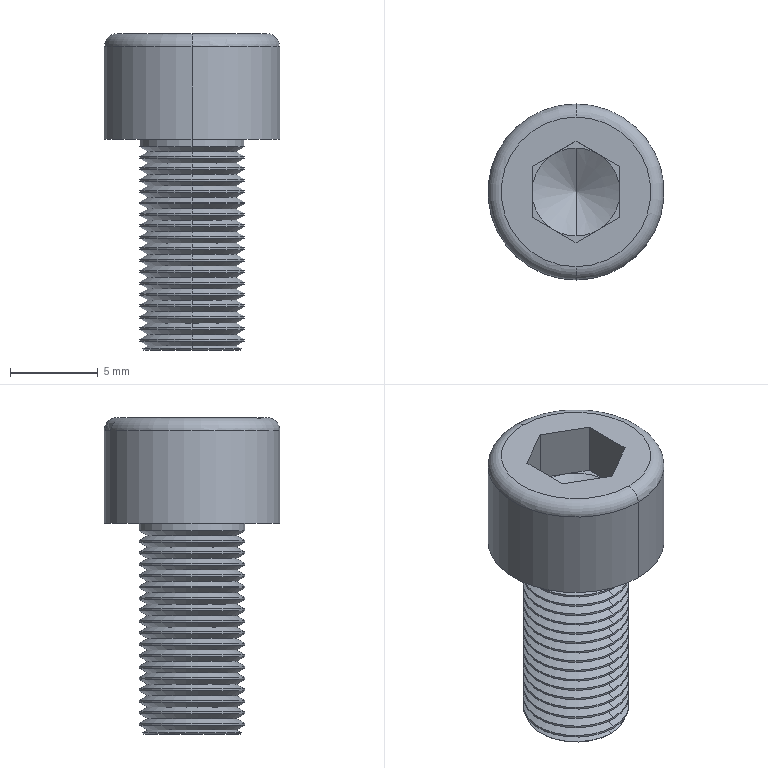Component | SolidWorks | LongSideClampingAssemblyBGeneralAssembly-1_HexagonSocketHeadCapScrew-M6X12-0510-1 | 1 solid | 131 faces | box 10 x 10 x 18 mm | volume 691 mm3 | cone 76 | cylinder 38 | plane 15 | torus 2 | commonest cylinder face diameters 6 x36 10 x2
build123d program:
from build123d import *

# Parameters (mm, degrees)
SKETCH1_R           = 5
BASEHEAD_DEPTH      = 6
SKETCH2_R           = 3
BASEBODY_DEPTH      = 12
HEXAGONSOCKET_DEPTH = 3
TOPFILLET_R         = 0.75
CHAMFER1_SIZE       = 0.25
LPATTERN10_COUNT    = 18
LPATTERN10_PITCH    = 0.6498


with BuildPart() as part:
    # Sketch1 → BaseHead (new body)
    with BuildSketch(Plane(origin=(0, 0, 0), x_dir=(0, 0, -1), z_dir=(1, 0, 0))):
        Circle(SKETCH1_R)
    extrude(amount=BASEHEAD_DEPTH)

    # Sketch2 → BaseBody (add)
    with BuildSketch(Plane(origin=(6, 0, 0), x_dir=(0, 0, -1), z_dir=(1, 0, 0))):
        Circle(SKETCH2_R)
    extrude(amount=BASEBODY_DEPTH)

    # Sketch3 → HexagonSocket (cut)
    with BuildSketch(Plane(origin=(0, 0, 0), x_dir=(0, 0, -1), z_dir=(1, 0, 0))):
        Polygon((2.887, 0), (1.443, 2.5), (-1.443, 2.5), (-2.887, 0), (-1.443, -2.5), (1.443, -2.5), align=None)
    extrude(amount=HEXAGONSOCKET_DEPTH, mode=Mode.SUBTRACT)

    # Sketch4 → Cut-Revolve1 (revolve, cut)
    with BuildSketch(Plane(origin=(-4.196, 0.75, 0), x_dir=(-1, 0, 0), z_dir=(0, 0, 1)), mode=Mode.PRIVATE) as cut_revolve1_sk:
        Polygon((-7.196, 3.25), (-8.64, 0.75), (-7.196, 0.75), align=None)
    revolve(cut_revolve1_sk.sketch.rotate(Axis((0.839, 0, 0), (-1, 0, 0)), 90), axis=Axis((0.839, 0, 0), (-1, 0, 0)), mode=Mode.SUBTRACT)

    # TopFillet
    topfillet_edges = [part.edges().sort_by_distance(p)[0] for p in [
        (0, 0, 5),
    ]]
    fillet(topfillet_edges, radius=TOPFILLET_R)

    # Chamfer1
    chamfer1_edges = [part.edges().sort_by_distance(p)[0] for p in [
        (18, 0, 3),
    ]]
    chamfer(chamfer1_edges, length=CHAMFER1_SIZE)

    # Sketch5 → Cut-Revolve10 (revolve, cut)
    with BuildSketch(Plane.XY, mode=Mode.PRIVATE) as cut_revolve10_sk:
        Polygon((17.75, 2.531), (18.021, 3), (18.021, 3.542), (17.479, 3.542), (17.479, 3), align=None)
    cut_revolve10 = revolve(cut_revolve10_sk.sketch.rotate(Axis((0, 0, 0), (1, 0, 0)), 90), axis=Axis((0, 0, 0), (1, 0, 0)), mode=Mode.SUBTRACT)

    # LPattern10: Cut-Revolve10 ×18
    with Locations(*[(-i * LPATTERN10_PITCH, 0, 0) for i in range(1, LPATTERN10_COUNT)]):
        add(cut_revolve10, mode=Mode.SUBTRACT)


solid = part.part

# Placed as in the assembly
solid = solid.moved(Location((-3081.658, -176.609, 3594.7), (90, 0, -90)))